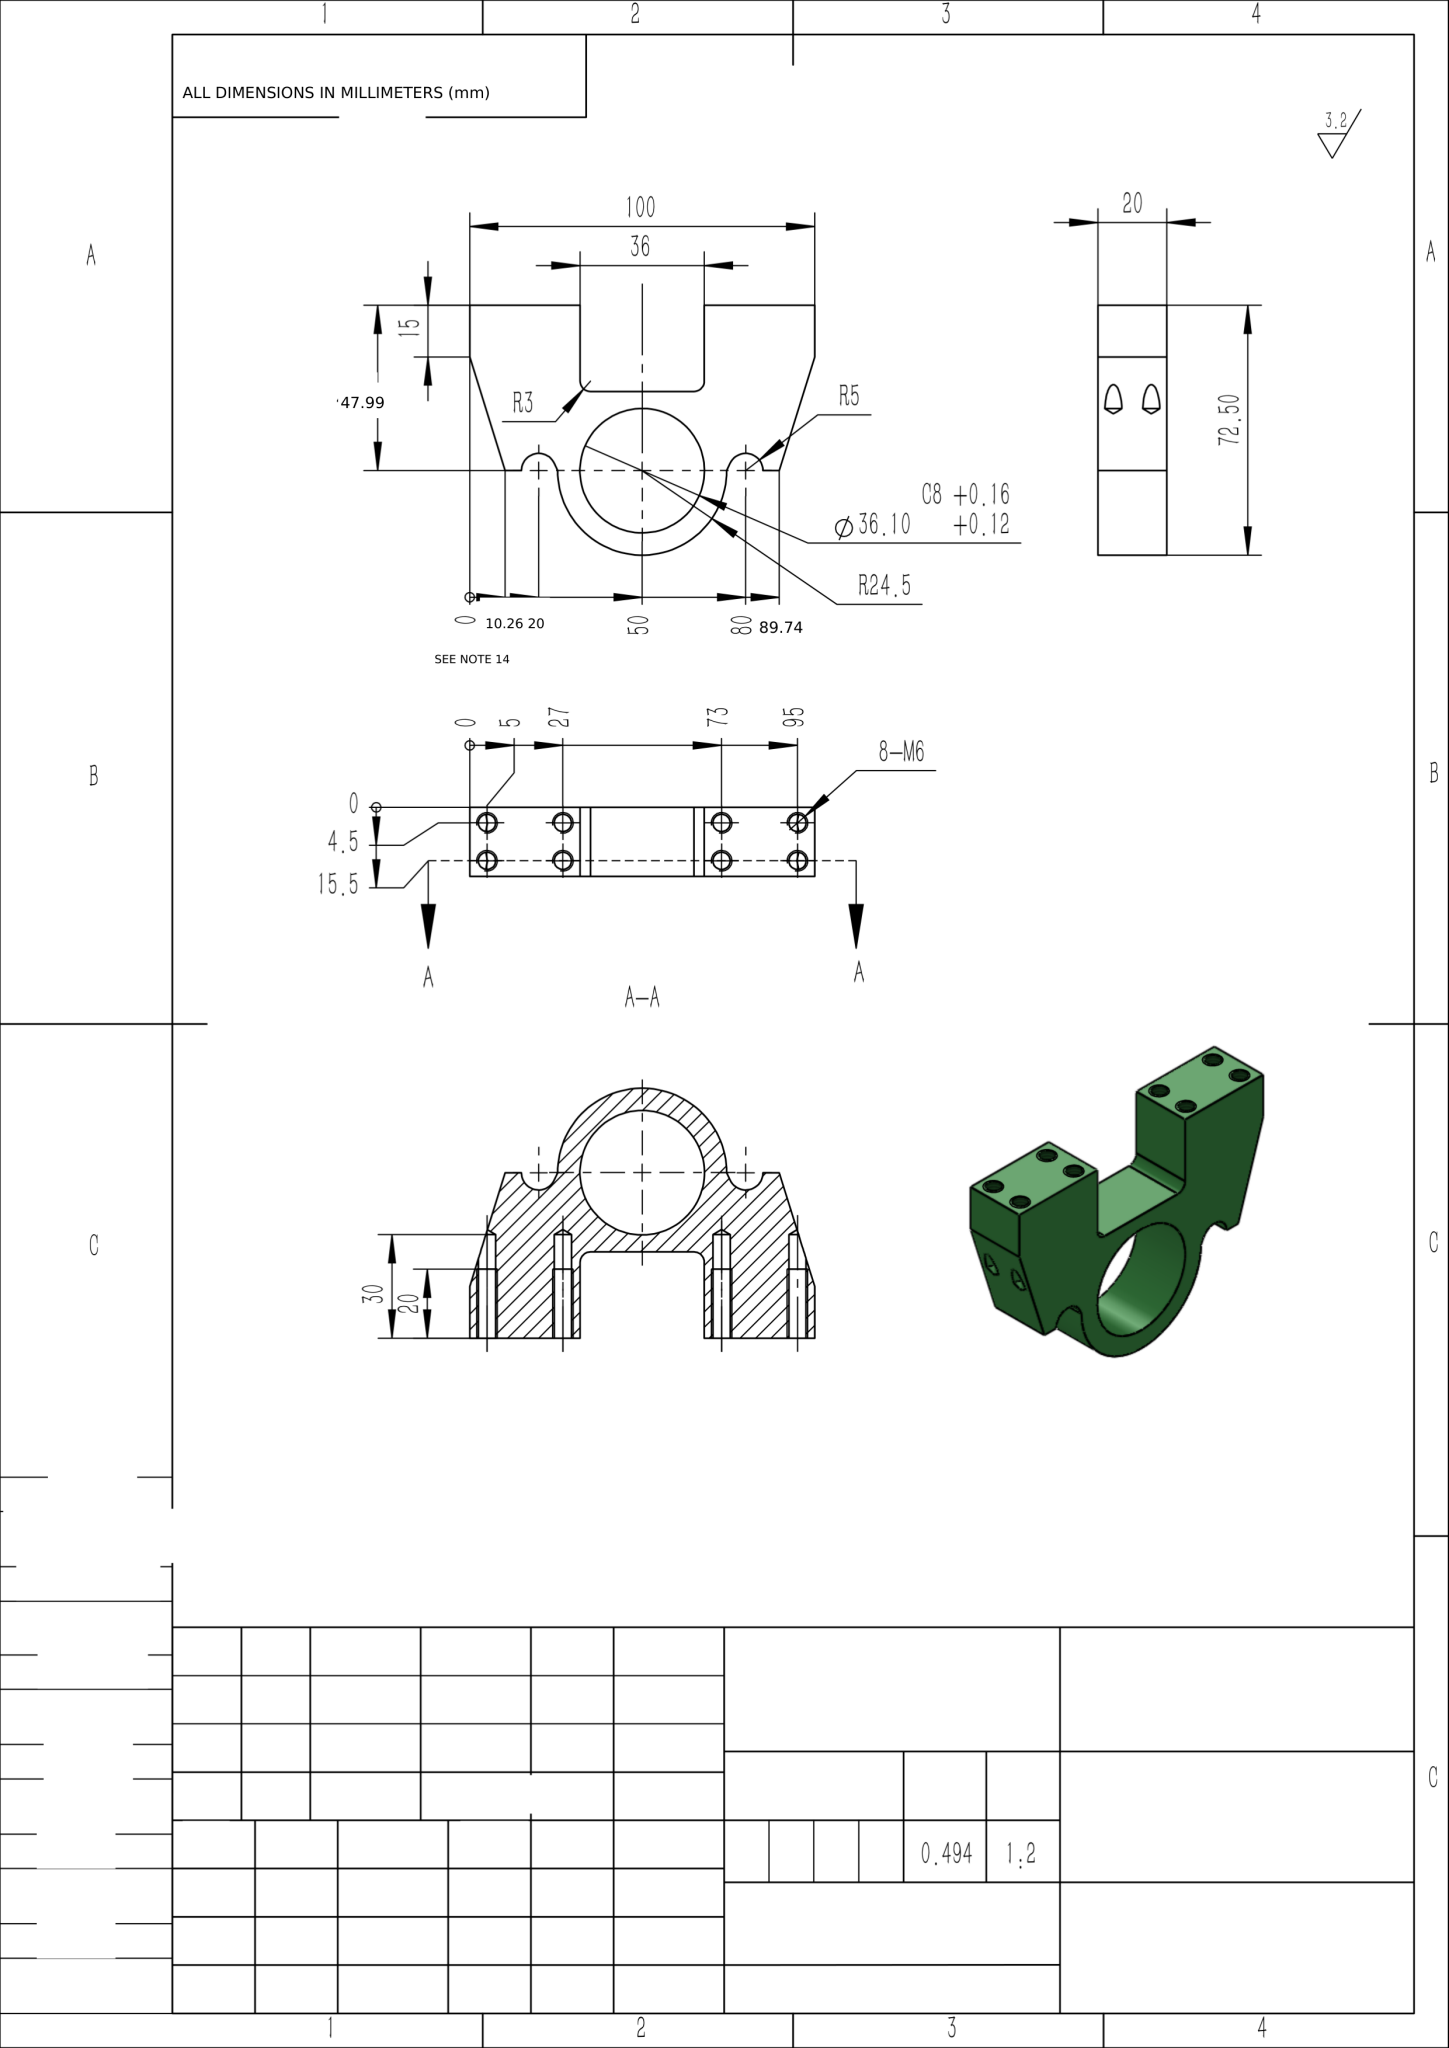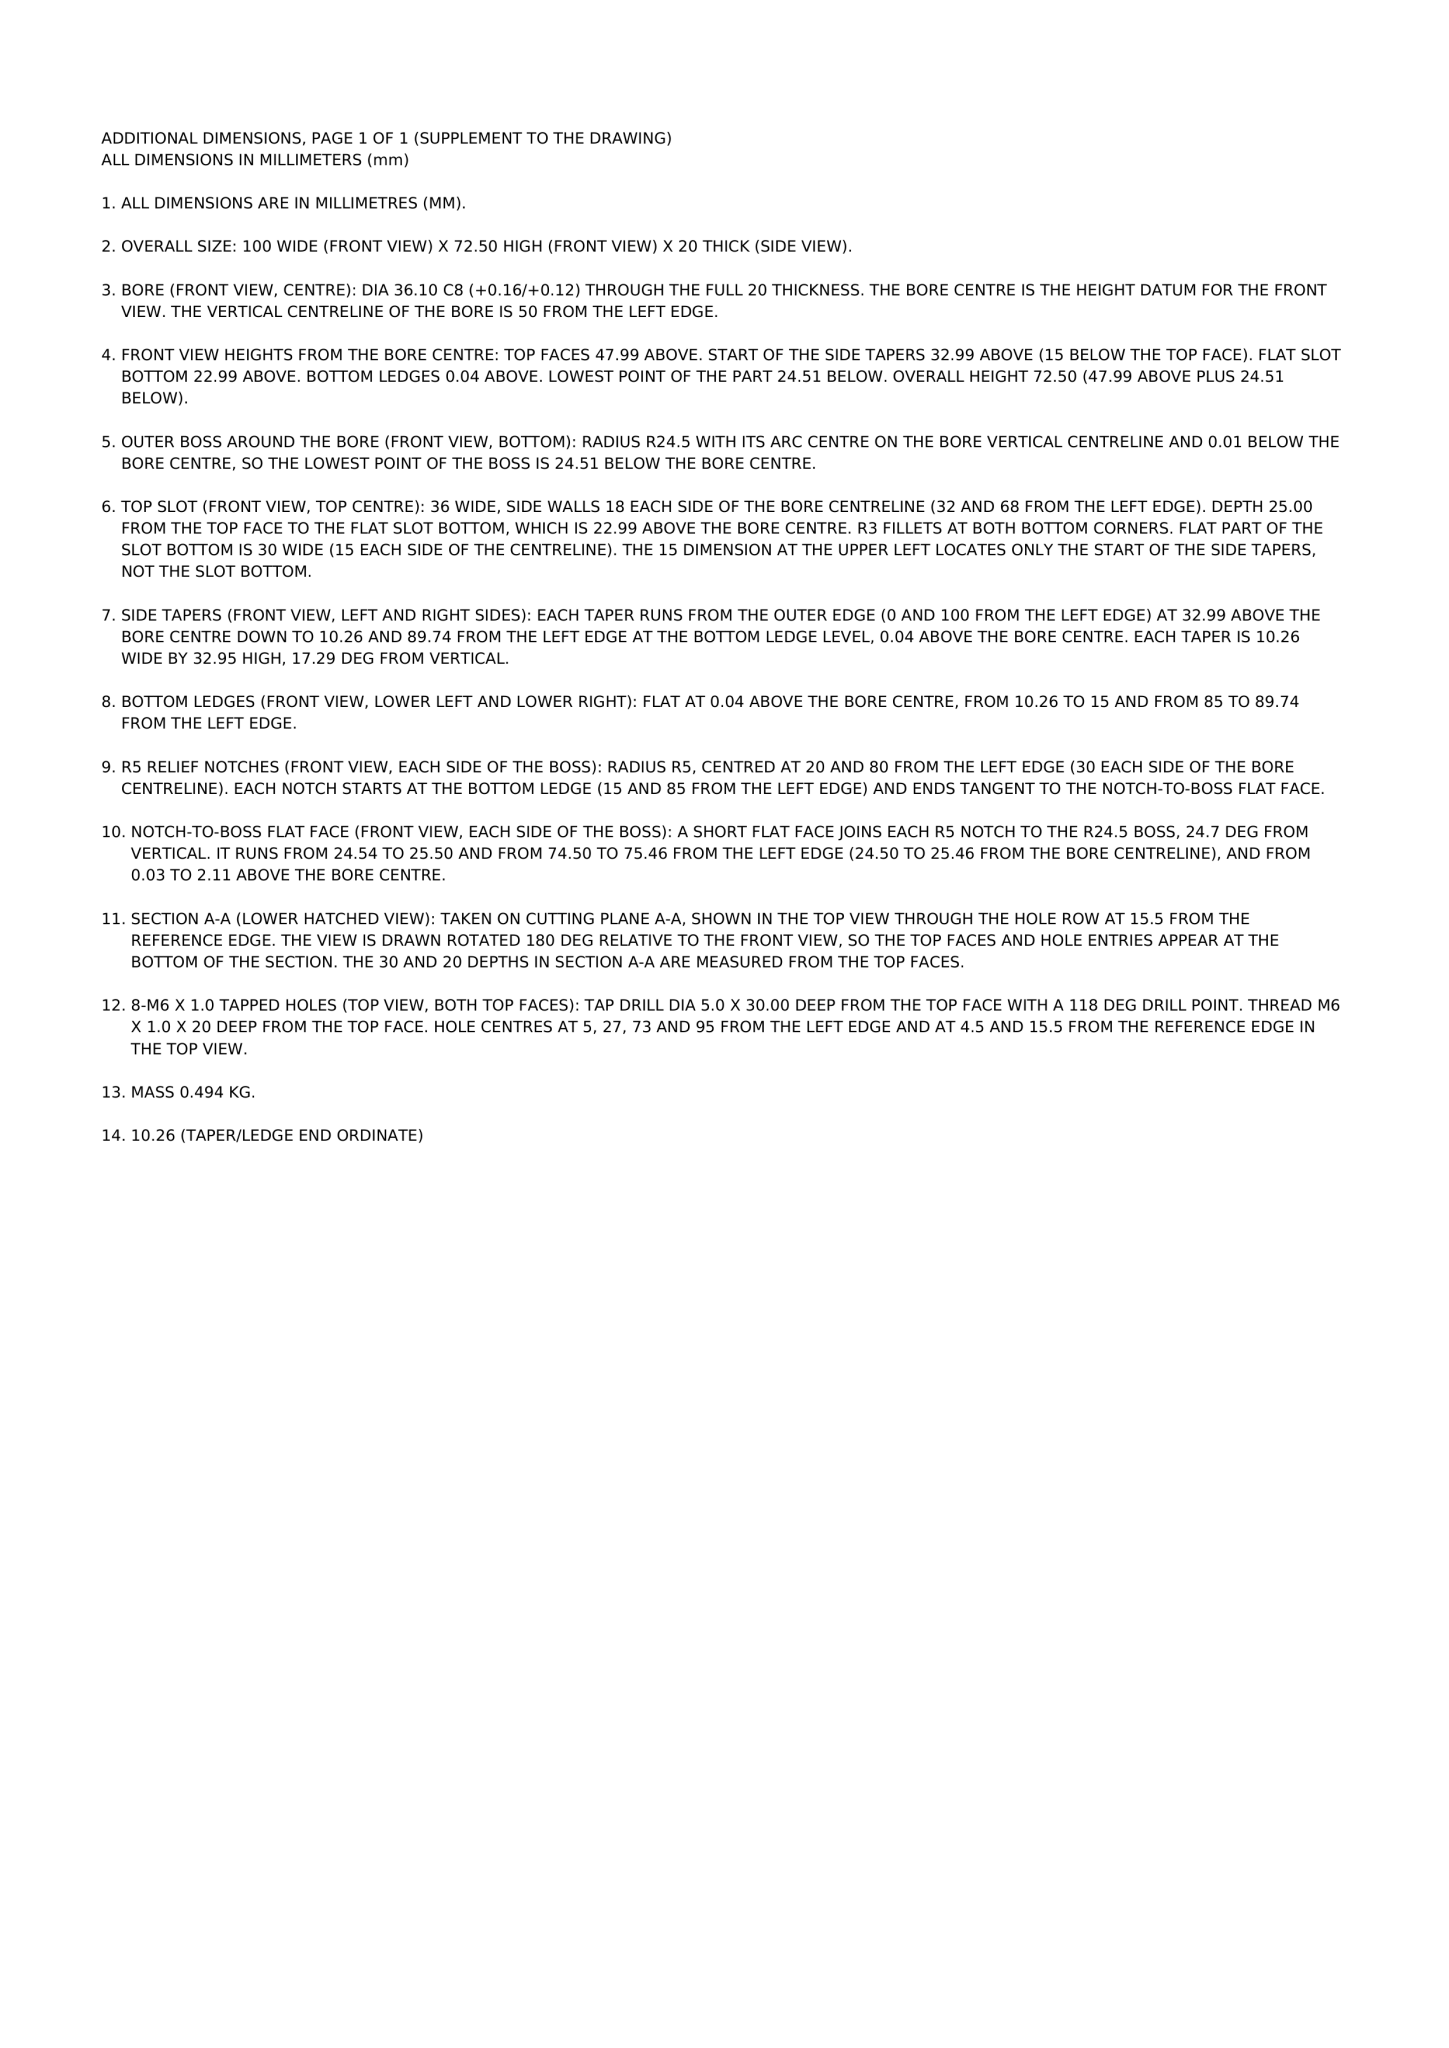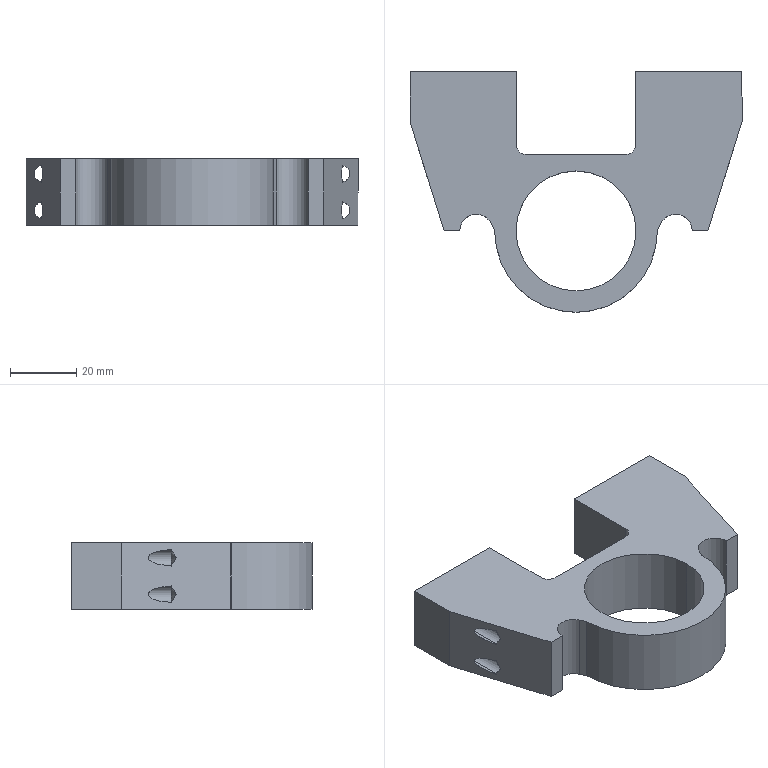Part | NX | mm | 1 solid | 60 faces | box 100 x 72.5 x 20 mm | volume 63395 mm3 | cylinder 25 | cone 20 | plane 15 | commonest cylinder face diameters 5 x16 49 x3 36.1 x2 6 x2 9.994 x2